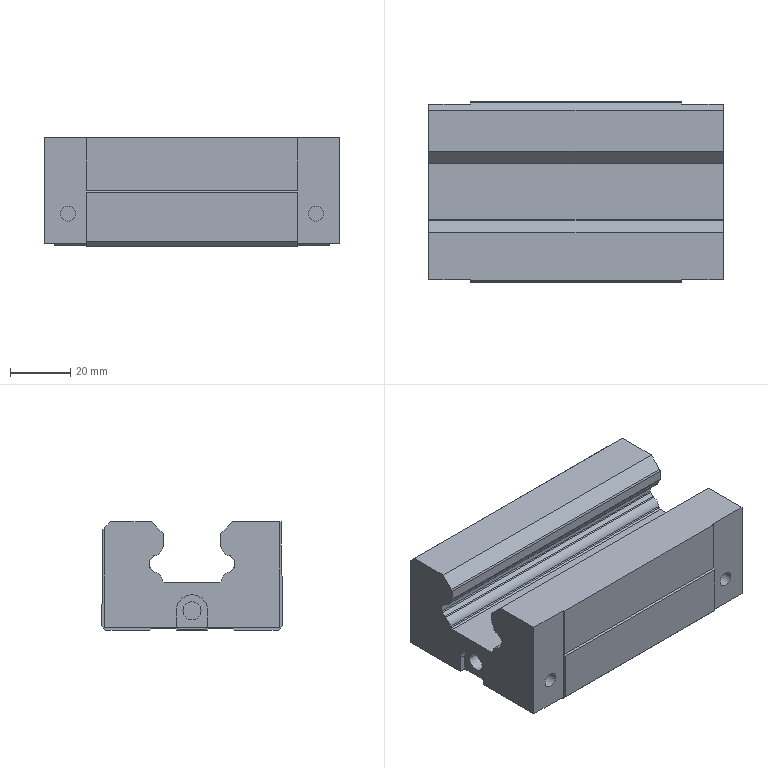Component | SolidWorks | SliderHGL30CA-2 | 1 solid | 132 faces | volume 157046 mm3 | plane 79 | cylinder 53 | commonest cylinder face diameters 1.2 x12 8 x8 5 x8 1 x7 6 x4 7.3 x4 5.66 x4 1.6 x4